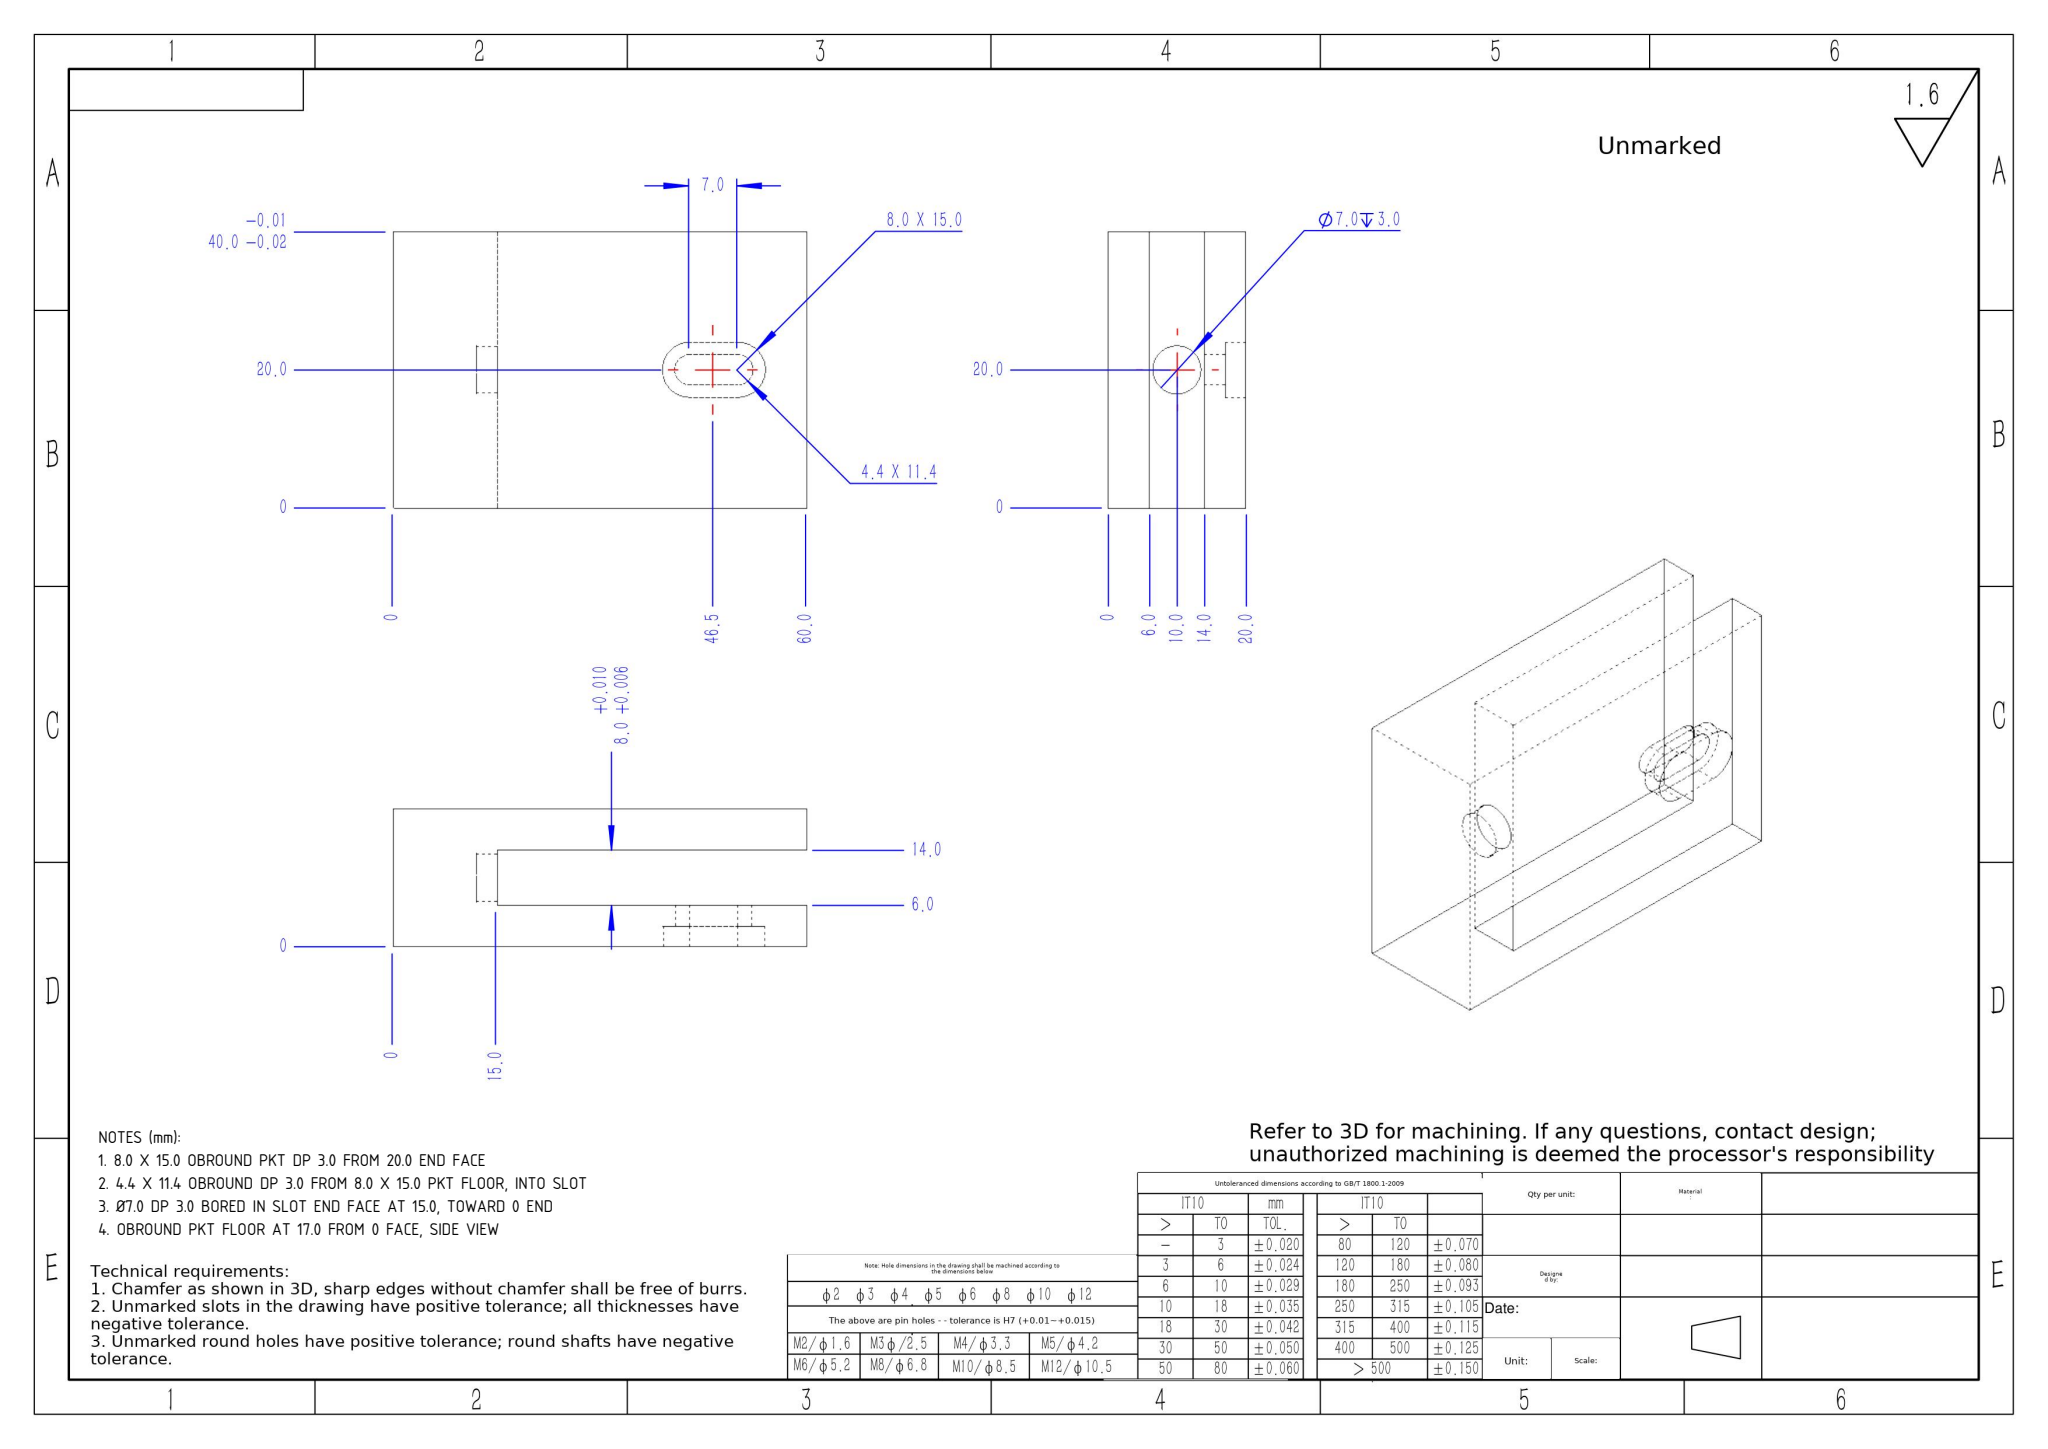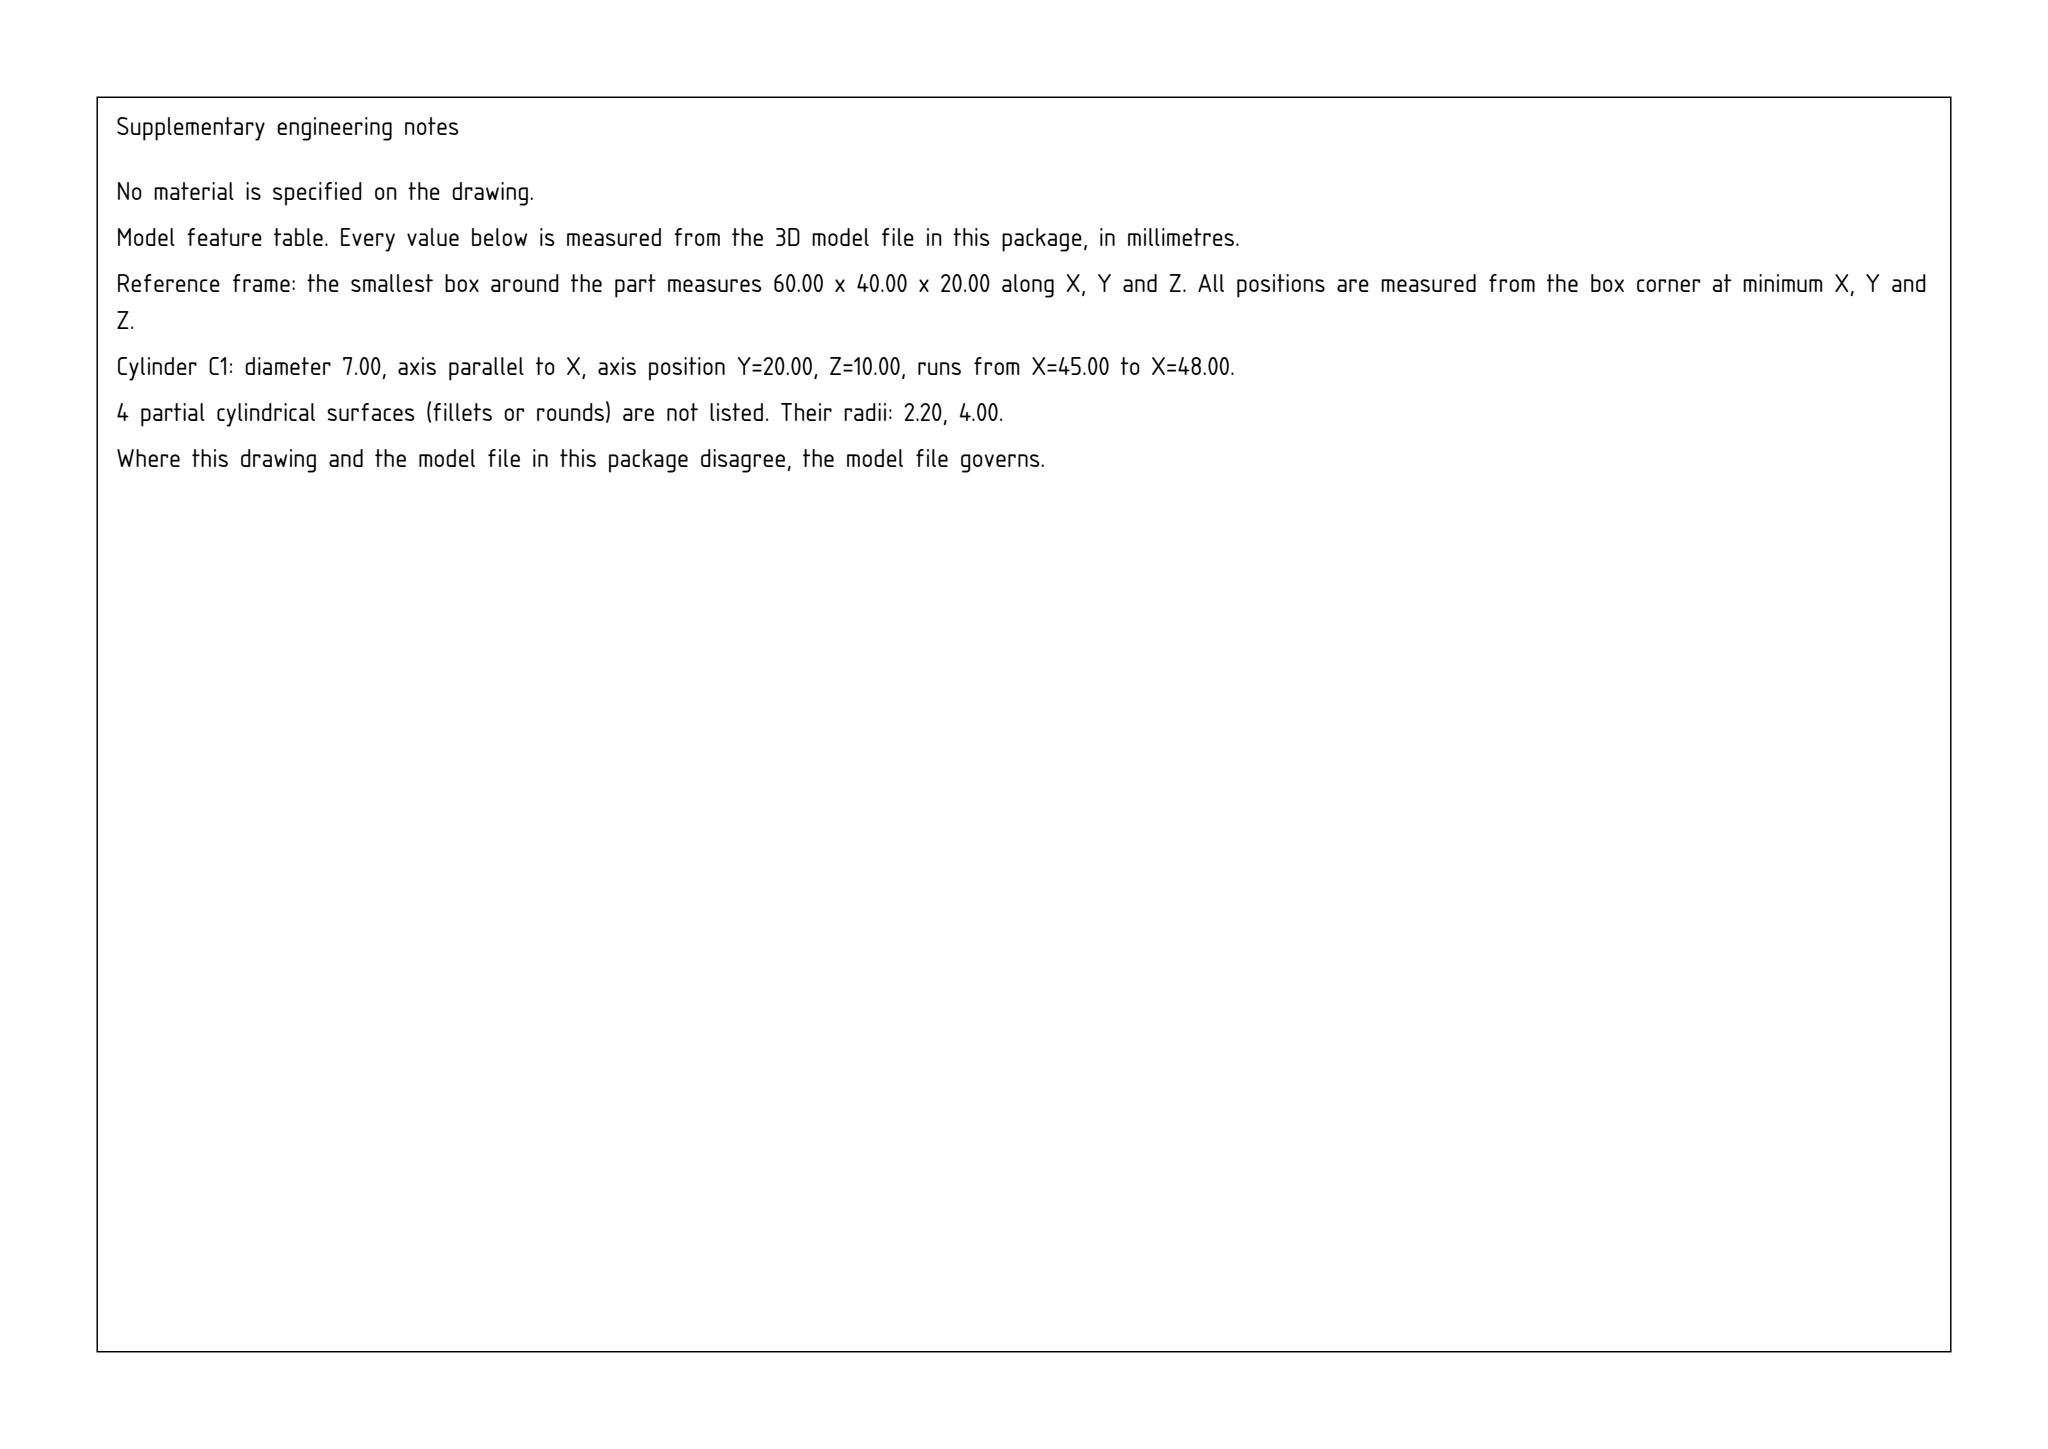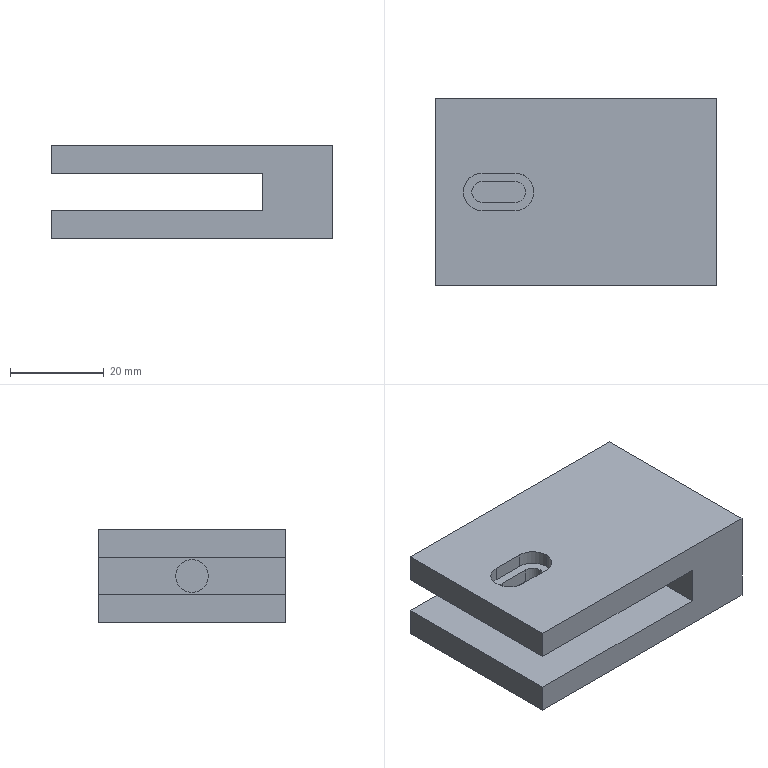Part | SolidWorks | mm | 1 solid | 24 faces | box 60 x 40 x 20 mm | volume 33028 mm3 | plane 16 | cylinder 8 | commonest cylinder face diameters 4.4 x3 8 x3 7 x2
Drawing notes:
8.0 X 15.0 OBROUND PKT DP 3.0 FROM 20.0 END FACE | from the solid: Ø8.0 z-axis cyls at x=10.0 & 17.0, y=20.0, len 3.0; z planes 20.0 & 17.0 (pocket 15.0 long overall = 7.0 ctr dist + 8.0)
4.4 X 11.4 OBROUND DP 3.0 FROM 8.0 X 15.0 PKT FLOOR, INTO SLOT | from the solid: Ø4.4 z-axis cyls at x=10.0 & 17.0, y=20.0, len 3.0; runs z=17.0 to z=14.0, breaking into slot (z planes 6.0/14.0); y planes 17.8/22.2
Ø7.0 DP 3.0 BORED IN SLOT END FACE AT 15.0, TOWARD 0 END | from the solid: Ø7.0 x-axis cyl, y=20.0, z=10.0, len 3.0; x planes 45.0 (slot end face = 15.0 in drawing) and 48.0 (bore btm)
OBROUND PKT FLOOR AT 17.0 FROM 0 FACE, SIDE VIEW | from the solid: z planes at 17.0 and 20.0; Ø8.0/Ø4.4 pocket cyls start at z=20.0 face, 3.0 deep
build123d program:
from build123d import *

# Parameters (mm, degrees)
SKETCH1_W           = 60
SKETCH1_H           = 40
BOSS_EXTRUDE1_DEPTH = 10
SKETCH2_W           = 45
SKETCH2_H           = 8
CUT_EXTRUDE1_DEPTH  = 51.99
CUT_EXTRUDE2_DEPTH  = 3
CUT_EXTRUDE3_DEPTH  = 3
SKETCH5_R           = 3.5
CUT_EXTRUDE4_DEPTH  = 3


with BuildPart() as part:
    # Sketch1 → Boss-Extrude1 (new, symmetric)
    with BuildSketch(Plane.XY):
        Rectangle(SKETCH1_W, SKETCH1_H)
    extrude(amount=BOSS_EXTRUDE1_DEPTH, both=True)

    # Sketch2 → Cut-Extrude1 (cut, through all)
    with BuildSketch(Plane(origin=(0, 20, 0), x_dir=(1, 0, 0), z_dir=(0, 1, 0))):
        with Locations((-7.5, 0)):
            Rectangle(SKETCH2_W, SKETCH2_H)
    extrude(amount=-CUT_EXTRUDE1_DEPTH, mode=Mode.SUBTRACT)

    # Sketch3 → Cut-Extrude2 (cut)
    with BuildSketch(Plane.XY.offset(10)):
        with BuildLine():
            Line((-20, 4), (-13, 4))
            ThreePointArc((-13, 4), (-9, 0), (-13, -4))
            Line((-13, -4), (-20, -4))
            ThreePointArc((-20, -4), (-24, 0), (-20, 4))
        make_face()
    extrude(amount=-CUT_EXTRUDE2_DEPTH, mode=Mode.SUBTRACT)

    # Sketch4 → Cut-Extrude3 (cut)
    with BuildSketch(Plane.XY.offset(7)):
        with BuildLine():
            Line((-20, 2.2), (-13, 2.2))
            ThreePointArc((-13, 2.2), (-10.8, 0), (-13, -2.2))
            Line((-13, -2.2), (-20, -2.2))
            ThreePointArc((-20, -2.2), (-22.2, 0), (-20, 2.2))
        make_face()
    extrude(amount=-CUT_EXTRUDE3_DEPTH, mode=Mode.SUBTRACT)

    # Sketch5 → Cut-Extrude4 (cut)
    with BuildSketch(Plane.ZY.offset(-15)):
        Circle(SKETCH5_R)
    extrude(amount=-CUT_EXTRUDE4_DEPTH, mode=Mode.SUBTRACT)


solid = part.part
STEP:
#1=CARTESIAN_POINT('',(18.,0.,-3.5));
#2=VERTEX_POINT('',#1);
#3=CARTESIAN_POINT('',(18.,0.,3.5));
#4=VERTEX_POINT('',#3);
#5=CARTESIAN_POINT('',(18.,0.,0.));
#6=DIRECTION('',(-1.,0.,0.));
#7=DIRECTION('',(0.,0.,1.));
#8=AXIS2_PLACEMENT_3D('',#5,#6,#7);
#9=CIRCLE('',#8,3.5);
#10=EDGE_CURVE('',#2,#4,#9,.T.);
#11=ORIENTED_EDGE('',*,*,#10,.F.);
#12=CARTESIAN_POINT('',(15.,0.,-3.5));
#13=VERTEX_POINT('',#12);
#14=CARTESIAN_POINT('',(18.,0.,-3.5));
#15=DIRECTION('',(-1.,0.,0.));
#16=VECTOR('',#15,1000.);
#17=LINE('',#14,#16);
#18=EDGE_CURVE('',#2,#13,#17,.T.);
#19=ORIENTED_EDGE('',*,*,#18,.T.);
#20=CARTESIAN_POINT('',(15.,0.,3.5));
#21=VERTEX_POINT('',#20);
#22=CARTESIAN_POINT('',(15.,0.,0.));
#23=DIRECTION('',(-1.,0.,0.));
#24=DIRECTION('',(0.,0.,1.));
#25=AXIS2_PLACEMENT_3D('',#22,#23,#24);
#26=CIRCLE('',#25,3.5);
#27=EDGE_CURVE('',#13,#21,#26,.T.);
#28=ORIENTED_EDGE('',*,*,#27,.T.);
#29=CARTESIAN_POINT('',(18.,0.,3.5));
#30=DIRECTION('',(-1.,0.,0.));
#31=VECTOR('',#30,1000.);
#32=LINE('',#29,#31);
#33=EDGE_CURVE('',#4,#21,#32,.T.);
#34=ORIENTED_EDGE('',*,*,#33,.F.);
#35=EDGE_LOOP('',(#11,#19,#28,#34));
#36=FACE_OUTER_BOUND('',#35,.T.);
#37=CARTESIAN_POINT('',(18.,0.,0.));
#38=DIRECTION('',(-1.,0.,0.));
#39=DIRECTION('',(0.,0.,1.));
#40=AXIS2_PLACEMENT_3D('',#37,#38,#39);
#41=CYLINDRICAL_SURFACE('',#40,3.5);
#42=ADVANCED_FACE('',(#36),#41,.F.);
#43=CARTESIAN_POINT('',(-10.8,0.,4.));
#44=VERTEX_POINT('',#43);
#45=CARTESIAN_POINT('',(-13.,2.2,4.));
#46=VERTEX_POINT('',#45);
#47=CARTESIAN_POINT('',(-13.,0.,4.));
#48=DIRECTION('',(0.,0.,1.));
#49=DIRECTION('',(1.,0.,0.));
#50=AXIS2_PLACEMENT_3D('',#47,#48,#49);
#51=CIRCLE('',#50,2.2);
#52=EDGE_CURVE('',#44,#46,#51,.T.);
#53=ORIENTED_EDGE('',*,*,#52,.F.);
#54=CARTESIAN_POINT('',(-10.8,0.,7.));
#55=VERTEX_POINT('',#54);
#56=CARTESIAN_POINT('',(-10.8,0.,4.));
#57=DIRECTION('',(0.,0.,1.));
#58=VECTOR('',#57,1000.);
#59=LINE('',#56,#58);
#60=EDGE_CURVE('',#44,#55,#59,.T.);
#61=ORIENTED_EDGE('',*,*,#60,.T.);
#62=CARTESIAN_POINT('',(-13.,2.2,7.));
#63=VERTEX_POINT('',#62);
#64=CARTESIAN_POINT('',(-13.,0.,7.));
#65=DIRECTION('',(0.,0.,1.));
#66=DIRECTION('',(1.,0.,0.));
#67=AXIS2_PLACEMENT_3D('',#64,#65,#66);
#68=CIRCLE('',#67,2.2);
#69=EDGE_CURVE('',#55,#63,#68,.T.);
#70=ORIENTED_EDGE('',*,*,#69,.T.);
#71=CARTESIAN_POINT('',(-13.,2.2,4.));
#72=DIRECTION('',(0.,0.,1.));
#73=VECTOR('',#72,1000.);
#74=LINE('',#71,#73);
#75=EDGE_CURVE('',#46,#63,#74,.T.);
#76=ORIENTED_EDGE('',*,*,#75,.F.);
#77=EDGE_LOOP('',(#53,#61,#70,#76));
#78=FACE_OUTER_BOUND('',#77,.T.);
#79=CARTESIAN_POINT('',(-13.,0.,4.));
#80=DIRECTION('',(0.,0.,1.));
#81=DIRECTION('',(1.,0.,0.));
#82=AXIS2_PLACEMENT_3D('',#79,#80,#81);
#83=CYLINDRICAL_SURFACE('',#82,2.2);
#84=ADVANCED_FACE('',(#78),#83,.F.);
#85=CARTESIAN_POINT('',(-9.,0.,7.));
#86=VERTEX_POINT('',#85);
#87=CARTESIAN_POINT('',(-13.,4.,7.));
#88=VERTEX_POINT('',#87);
#89=CARTESIAN_POINT('',(-13.,0.,7.));
#90=DIRECTION('',(0.,0.,1.));
#91=DIRECTION('',(1.,0.,0.));
#92=AXIS2_PLACEMENT_3D('',#89,#90,#91);
#93=CIRCLE('',#92,4.);
#94=EDGE_CURVE('',#86,#88,#93,.T.);
#95=ORIENTED_EDGE('',*,*,#94,.F.);
#96=CARTESIAN_POINT('',(-9.,0.,10.));
#97=VERTEX_POINT('',#96);
#98=CARTESIAN_POINT('',(-9.,0.,7.));
#99=DIRECTION('',(0.,0.,1.));
#100=VECTOR('',#99,1000.);
#101=LINE('',#98,#100);
#102=EDGE_CURVE('',#86,#97,#101,.T.);
#103=ORIENTED_EDGE('',*,*,#102,.T.);
#104=CARTESIAN_POINT('',(-13.,4.,10.));
#105=VERTEX_POINT('',#104);
#106=CARTESIAN_POINT('',(-13.,0.,10.));
#107=DIRECTION('',(0.,0.,1.));
#108=DIRECTION('',(1.,0.,0.));
#109=AXIS2_PLACEMENT_3D('',#106,#107,#108);
#110=CIRCLE('',#109,4.);
#111=EDGE_CURVE('',#97,#105,#110,.T.);
#112=ORIENTED_EDGE('',*,*,#111,.T.);
#113=CARTESIAN_POINT('',(-13.,4.,7.));
#114=DIRECTION('',(0.,0.,1.));
#115=VECTOR('',#114,1000.);
#116=LINE('',#113,#115);
#117=EDGE_CURVE('',#88,#105,#116,.T.);
#118=ORIENTED_EDGE('',*,*,#117,.F.);
#119=EDGE_LOOP('',(#95,#103,#112,#118));
#120=FACE_OUTER_BOUND('',#119,.T.);
#121=CARTESIAN_POINT('',(-13.,0.,7.));
#122=DIRECTION('',(0.,0.,1.));
#123=DIRECTION('',(1.,0.,0.));
#124=AXIS2_PLACEMENT_3D('',#121,#122,#123);
#125=CYLINDRICAL_SURFACE('',#124,4.);
#126=ADVANCED_FACE('',(#120),#125,.F.);
#127=CARTESIAN_POINT('',(-30.,-20.,-4.));
#128=VERTEX_POINT('',#127);
#129=CARTESIAN_POINT('',(-30.,-20.,-10.));
#130=VERTEX_POINT('',#129);
#131=CARTESIAN_POINT('',(-30.,-20.,10.));
#132=DIRECTION('',(0.,0.,-1.));
#133=VECTOR('',#132,1000.);
#134=LINE('',#131,#133);
#135=EDGE_CURVE('',#128,#130,#134,.T.);
#136=ORIENTED_EDGE('',*,*,#135,.F.);
#137=CARTESIAN_POINT('',(-30.,20.,-4.));
#138=VERTEX_POINT('',#137);
#139=CARTESIAN_POINT('',(-30.,-20.,-4.));
#140=DIRECTION('',(0.,1.,0.));
#141=VECTOR('',#140,1000.);
#142=LINE('',#139,#141);
#143=EDGE_CURVE('',#128,#138,#142,.T.);
#144=ORIENTED_EDGE('',*,*,#143,.T.);
#145=CARTESIAN_POINT('',(-30.,20.,-10.));
#146=VERTEX_POINT('',#145);
#147=CARTESIAN_POINT('',(-30.,20.,10.));
#148=DIRECTION('',(0.,0.,-1.));
#149=VECTOR('',#148,1000.);
#150=LINE('',#147,#149);
#151=EDGE_CURVE('',#138,#146,#150,.T.);
#152=ORIENTED_EDGE('',*,*,#151,.T.);
#153=CARTESIAN_POINT('',(-30.,-20.,-10.));
#154=DIRECTION('',(0.,-1.,0.));
#155=VECTOR('',#154,1000.);
#156=LINE('',#153,#155);
#157=EDGE_CURVE('',#146,#130,#156,.T.);
#158=ORIENTED_EDGE('',*,*,#157,.T.);
#159=EDGE_LOOP('',(#136,#144,#152,#158));
#160=FACE_OUTER_BOUND('',#159,.T.);
#161=CARTESIAN_POINT('',(-30.,-20.,10.));
#162=DIRECTION('',(1.,0.,0.));
#163=DIRECTION('',(0.,0.,-1.));
#164=AXIS2_PLACEMENT_3D('',#161,#162,#163);
#165=PLANE('',#164);
#166=ADVANCED_FACE('',(#160),#165,.F.);
#167=CARTESIAN_POINT('',(-30.,20.,10.));
#168=VERTEX_POINT('',#167);
#169=CARTESIAN_POINT('',(-30.,20.,4.));
#170=VERTEX_POINT('',#169);
#171=CARTESIAN_POINT('',(-30.,20.,10.));
#172=DIRECTION('',(0.,0.,-1.));
#173=VECTOR('',#172,1000.);
#174=LINE('',#171,#173);
#175=EDGE_CURVE('',#168,#170,#174,.T.);
#176=ORIENTED_EDGE('',*,*,#175,.T.);
#177=CARTESIAN_POINT('',(-30.,-20.,4.));
#178=VERTEX_POINT('',#177);
#179=CARTESIAN_POINT('',(-30.,-20.,4.));
#180=DIRECTION('',(0.,1.,0.));
#181=VECTOR('',#180,1000.);
#182=LINE('',#179,#181);
#183=EDGE_CURVE('',#178,#170,#182,.T.);
#184=ORIENTED_EDGE('',*,*,#183,.F.);
#185=CARTESIAN_POINT('',(-30.,-20.,10.));
#186=VERTEX_POINT('',#185);
#187=CARTESIAN_POINT('',(-30.,-20.,10.));
#188=DIRECTION('',(0.,0.,-1.));
#189=VECTOR('',#188,1000.);
#190=LINE('',#187,#189);
#191=EDGE_CURVE('',#186,#178,#190,.T.);
#192=ORIENTED_EDGE('',*,*,#191,.F.);
#193=CARTESIAN_POINT('',(-30.,-20.,10.));
#194=DIRECTION('',(0.,-1.,0.));
#195=VECTOR('',#194,1000.);
#196=LINE('',#193,#195);
#197=EDGE_CURVE('',#168,#186,#196,.T.);
#198=ORIENTED_EDGE('',*,*,#197,.F.);
#199=EDGE_LOOP('',(#176,#184,#192,#198));
#200=FACE_OUTER_BOUND('',#199,.T.);
#201=CARTESIAN_POINT('',(-30.,-20.,10.));
#202=DIRECTION('',(1.,0.,0.));
#203=DIRECTION('',(0.,0.,-1.));
#204=AXIS2_PLACEMENT_3D('',#201,#202,#203);
#205=PLANE('',#204);
#206=ADVANCED_FACE('',(#200),#205,.F.);
#207=CARTESIAN_POINT('',(15.,-20.,4.));
#208=VERTEX_POINT('',#207);
#209=CARTESIAN_POINT('',(15.,-20.,-4.));
#210=VERTEX_POINT('',#209);
#211=CARTESIAN_POINT('',(15.,-20.,-4.));
#212=DIRECTION('',(0.,0.,-1.));
#213=VECTOR('',#212,1000.);
#214=LINE('',#211,#213);
#215=EDGE_CURVE('',#208,#210,#214,.T.);
#216=ORIENTED_EDGE('',*,*,#215,.T.);
#217=CARTESIAN_POINT('',(-30.,-20.,-4.));
#218=DIRECTION('',(-1.,0.,0.));
#219=VECTOR('',#218,1000.);
#220=LINE('',#217,#219);
#221=EDGE_CURVE('',#210,#128,#220,.T.);
#222=ORIENTED_EDGE('',*,*,#221,.T.);
#223=ORIENTED_EDGE('',*,*,#135,.T.);
#224=CARTESIAN_POINT('',(30.,-20.,-10.));
#225=VERTEX_POINT('',#224);
#226=CARTESIAN_POINT('',(30.,-20.,-10.));
#227=DIRECTION('',(1.,-0.,0.));
#228=VECTOR('',#227,1000.);
#229=LINE('',#226,#228);
#230=EDGE_CURVE('',#130,#225,#229,.T.);
#231=ORIENTED_EDGE('',*,*,#230,.T.);
#232=CARTESIAN_POINT('',(30.,-20.,10.));
#233=VERTEX_POINT('',#232);
#234=CARTESIAN_POINT('',(30.,-20.,10.));
#235=DIRECTION('',(0.,0.,-1.));
#236=VECTOR('',#235,1000.);
#237=LINE('',#234,#236);
#238=EDGE_CURVE('',#233,#225,#237,.T.);
#239=ORIENTED_EDGE('',*,*,#238,.F.);
#240=CARTESIAN_POINT('',(30.,-20.,10.));
#241=DIRECTION('',(1.,-0.,0.));
#242=VECTOR('',#241,1000.);
#243=LINE('',#240,#242);
#244=EDGE_CURVE('',#186,#233,#243,.T.);
#245=ORIENTED_EDGE('',*,*,#244,.F.);
#246=ORIENTED_EDGE('',*,*,#191,.T.);
#247=CARTESIAN_POINT('',(-30.,-20.,4.));
#248=DIRECTION('',(1.,0.,0.));
#249=VECTOR('',#248,1000.);
#250=LINE('',#247,#249);
#251=EDGE_CURVE('',#178,#208,#250,.T.);
#252=ORIENTED_EDGE('',*,*,#251,.T.);
#253=EDGE_LOOP('',(#216,#222,#223,#231,#239,#245,#246,#252));
#254=FACE_OUTER_BOUND('',#253,.T.);
#255=CARTESIAN_POINT('',(30.,-20.,10.));
#256=DIRECTION('',(0.,1.,0.));
#257=DIRECTION('',(-1.,0.,0.));
#258=AXIS2_PLACEMENT_3D('',#255,#256,#257);
#259=PLANE('',#258);
#260=ADVANCED_FACE('',(#254),#259,.F.);
#261=CARTESIAN_POINT('',(30.,20.,-10.));
#262=VERTEX_POINT('',#261);
#263=CARTESIAN_POINT('',(30.,-20.,-10.));
#264=DIRECTION('',(-0.,1.,0.));
#265=VECTOR('',#264,1000.);
#266=LINE('',#263,#265);
#267=EDGE_CURVE('',#225,#262,#266,.T.);
#268=ORIENTED_EDGE('',*,*,#267,.T.);
#269=CARTESIAN_POINT('',(30.,20.,10.));
#270=VERTEX_POINT('',#269);
#271=CARTESIAN_POINT('',(30.,20.,10.));
#272=DIRECTION('',(0.,0.,-1.));
#273=VECTOR('',#272,1000.);
#274=LINE('',#271,#273);
#275=EDGE_CURVE('',#270,#262,#274,.T.);
#276=ORIENTED_EDGE('',*,*,#275,.F.);
#277=CARTESIAN_POINT('',(30.,-20.,10.));
#278=DIRECTION('',(-0.,1.,0.));
#279=VECTOR('',#278,1000.);
#280=LINE('',#277,#279);
#281=EDGE_CURVE('',#233,#270,#280,.T.);
#282=ORIENTED_EDGE('',*,*,#281,.F.);
#283=ORIENTED_EDGE('',*,*,#238,.T.);
#284=EDGE_LOOP('',(#268,#276,#282,#283));
#285=FACE_OUTER_BOUND('',#284,.T.);
#286=CARTESIAN_POINT('',(30.,-20.,10.));
#287=DIRECTION('',(-1.,-0.,0.));
#288=DIRECTION('',(0.,-1.,0.));
#289=AXIS2_PLACEMENT_3D('',#286,#287,#288);
#290=PLANE('',#289);
#291=ADVANCED_FACE('',(#285),#290,.F.);
#292=ORIENTED_EDGE('',*,*,#151,.F.);
#293=CARTESIAN_POINT('',(15.,20.,-4.));
#294=VERTEX_POINT('',#293);
#295=CARTESIAN_POINT('',(-30.,20.,-4.));
#296=DIRECTION('',(-1.,0.,0.));
#297=VECTOR('',#296,1000.);
#298=LINE('',#295,#297);
#299=EDGE_CURVE('',#294,#138,#298,.T.);
#300=ORIENTED_EDGE('',*,*,#299,.F.);
#301=CARTESIAN_POINT('',(15.,20.,4.));
#302=VERTEX_POINT('',#301);
#303=CARTESIAN_POINT('',(15.,20.,-4.));
#304=DIRECTION('',(0.,0.,-1.));
#305=VECTOR('',#304,1000.);
#306=LINE('',#303,#305);
#307=EDGE_CURVE('',#302,#294,#306,.T.);
#308=ORIENTED_EDGE('',*,*,#307,.F.);
#309=CARTESIAN_POINT('',(-30.,20.,4.));
#310=DIRECTION('',(1.,0.,0.));
#311=VECTOR('',#310,1000.);
#312=LINE('',#309,#311);
#313=EDGE_CURVE('',#170,#302,#312,.T.);
#314=ORIENTED_EDGE('',*,*,#313,.F.);
#315=ORIENTED_EDGE('',*,*,#175,.F.);
#316=CARTESIAN_POINT('',(30.,20.,10.));
#317=DIRECTION('',(-1.,0.,0.));
#318=VECTOR('',#317,1000.);
#319=LINE('',#316,#318);
#320=EDGE_CURVE('',#270,#168,#319,.T.);
#321=ORIENTED_EDGE('',*,*,#320,.F.);
#322=ORIENTED_EDGE('',*,*,#275,.T.);
#323=CARTESIAN_POINT('',(30.,20.,-10.));
#324=DIRECTION('',(-1.,0.,0.));
#325=VECTOR('',#324,1000.);
#326=LINE('',#323,#325);
#327=EDGE_CURVE('',#262,#146,#326,.T.);
#328=ORIENTED_EDGE('',*,*,#327,.T.);
#329=EDGE_LOOP('',(#292,#300,#308,#314,#315,#321,#322,#328));
#330=FACE_OUTER_BOUND('',#329,.T.);
#331=CARTESIAN_POINT('',(30.,20.,10.));
#332=DIRECTION('',(0.,-1.,0.));
#333=DIRECTION('',(0.,0.,-1.));
#334=AXIS2_PLACEMENT_3D('',#331,#332,#333);
#335=PLANE('',#334);
#336=ADVANCED_FACE('',(#330),#335,.F.);
#337=CARTESIAN_POINT('',(-20.,4.,10.));
#338=VERTEX_POINT('',#337);
#339=CARTESIAN_POINT('',(-20.,-4.,10.));
#340=VERTEX_POINT('',#339);
#341=CARTESIAN_POINT('',(-20.,0.,10.));
#342=DIRECTION('',(0.,0.,1.));
#343=DIRECTION('',(1.,0.,0.));
#344=AXIS2_PLACEMENT_3D('',#341,#342,#343);
#345=CIRCLE('',#344,4.);
#346=EDGE_CURVE('',#338,#340,#345,.T.);
#347=ORIENTED_EDGE('',*,*,#346,.F.);
#348=CARTESIAN_POINT('',(-20.,4.,10.));
#349=DIRECTION('',(-1.,0.,0.));
#350=VECTOR('',#349,1000.);
#351=LINE('',#348,#350);
#352=EDGE_CURVE('',#105,#338,#351,.T.);
#353=ORIENTED_EDGE('',*,*,#352,.F.);
#354=ORIENTED_EDGE('',*,*,#111,.F.);
#355=CARTESIAN_POINT('',(-13.,-4.,10.));
#356=VERTEX_POINT('',#355);
#357=CARTESIAN_POINT('',(-13.,0.,10.));
#358=DIRECTION('',(0.,0.,1.));
#359=DIRECTION('',(1.,0.,0.));
#360=AXIS2_PLACEMENT_3D('',#357,#358,#359);
#361=CIRCLE('',#360,4.);
#362=EDGE_CURVE('',#356,#97,#361,.T.);
#363=ORIENTED_EDGE('',*,*,#362,.F.);
#364=CARTESIAN_POINT('',(-20.,-4.,10.));
#365=DIRECTION('',(1.,0.,0.));
#366=VECTOR('',#365,1000.);
#367=LINE('',#364,#366);
#368=EDGE_CURVE('',#340,#356,#367,.T.);
#369=ORIENTED_EDGE('',*,*,#368,.F.);
#370=EDGE_LOOP('',(#347,#353,#354,#363,#369));
#371=FACE_BOUND('',#370,.T.);
#372=ORIENTED_EDGE('',*,*,#197,.T.);
#373=ORIENTED_EDGE('',*,*,#244,.T.);
#374=ORIENTED_EDGE('',*,*,#281,.T.);
#375=ORIENTED_EDGE('',*,*,#320,.T.);
#376=EDGE_LOOP('',(#372,#373,#374,#375));
#377=FACE_OUTER_BOUND('',#376,.T.);
#378=CARTESIAN_POINT('',(0.,0.,10.));
#379=DIRECTION('',(0.,0.,1.));
#380=DIRECTION('',(1.,0.,0.));
#381=AXIS2_PLACEMENT_3D('',#378,#379,#380);
#382=PLANE('',#381);
#383=ADVANCED_FACE('',(#371,#377),#382,.T.);
#384=ORIENTED_EDGE('',*,*,#157,.F.);
#385=ORIENTED_EDGE('',*,*,#327,.F.);
#386=ORIENTED_EDGE('',*,*,#267,.F.);
#387=ORIENTED_EDGE('',*,*,#230,.F.);
#388=EDGE_LOOP('',(#384,#385,#386,#387));
#389=FACE_OUTER_BOUND('',#388,.T.);
#390=CARTESIAN_POINT('',(0.,0.,-10.));
#391=DIRECTION('',(0.,0.,1.));
#392=DIRECTION('',(1.,0.,0.));
#393=AXIS2_PLACEMENT_3D('',#390,#391,#392);
#394=PLANE('',#393);
#395=ADVANCED_FACE('',(#389),#394,.F.);
#396=ORIENTED_EDGE('',*,*,#299,.T.);
#397=ORIENTED_EDGE('',*,*,#143,.F.);
#398=ORIENTED_EDGE('',*,*,#221,.F.);
#399=CARTESIAN_POINT('',(15.,-20.,-4.));
#400=DIRECTION('',(0.,1.,0.));
#401=VECTOR('',#400,1000.);
#402=LINE('',#399,#401);
#403=EDGE_CURVE('',#210,#294,#402,.T.);
#404=ORIENTED_EDGE('',*,*,#403,.T.);
#405=EDGE_LOOP('',(#396,#397,#398,#404));
#406=FACE_OUTER_BOUND('',#405,.T.);
#407=CARTESIAN_POINT('',(-30.,-20.,-4.));
#408=DIRECTION('',(0.,0.,-1.));
#409=DIRECTION('',(-1.,0.,0.));
#410=AXIS2_PLACEMENT_3D('',#407,#408,#409);
#411=PLANE('',#410);
#412=ADVANCED_FACE('',(#406),#411,.F.);
#413=CARTESIAN_POINT('',(15.,0.,0.));
#414=DIRECTION('',(-1.,0.,0.));
#415=DIRECTION('',(0.,0.,1.));
#416=AXIS2_PLACEMENT_3D('',#413,#414,#415);
#417=CIRCLE('',#416,3.5);
#418=EDGE_CURVE('',#21,#13,#417,.T.);
#419=ORIENTED_EDGE('',*,*,#418,.F.);
#420=ORIENTED_EDGE('',*,*,#27,.F.);
#421=EDGE_LOOP('',(#419,#420));
#422=FACE_BOUND('',#421,.T.);
#423=ORIENTED_EDGE('',*,*,#307,.T.);
#424=ORIENTED_EDGE('',*,*,#403,.F.);
#425=ORIENTED_EDGE('',*,*,#215,.F.);
#426=CARTESIAN_POINT('',(15.,-20.,4.));
#427=DIRECTION('',(0.,1.,0.));
#428=VECTOR('',#427,1000.);
#429=LINE('',#426,#428);
#430=EDGE_CURVE('',#208,#302,#429,.T.);
#431=ORIENTED_EDGE('',*,*,#430,.T.);
#432=EDGE_LOOP('',(#423,#424,#425,#431));
#433=FACE_OUTER_BOUND('',#432,.T.);
#434=CARTESIAN_POINT('',(15.,-20.,-4.));
#435=DIRECTION('',(1.,0.,0.));
#436=DIRECTION('',(0.,0.,-1.));
#437=AXIS2_PLACEMENT_3D('',#434,#435,#436);
#438=PLANE('',#437);
#439=ADVANCED_FACE('',(#422,#433),#438,.F.);
#440=CARTESIAN_POINT('',(-20.,2.2,4.));
#441=VERTEX_POINT('',#440);
#442=CARTESIAN_POINT('',(-20.,2.2,4.));
#443=DIRECTION('',(-1.,0.,0.));
#444=VECTOR('',#443,1000.);
#445=LINE('',#442,#444);
#446=EDGE_CURVE('',#46,#441,#445,.T.);
#447=ORIENTED_EDGE('',*,*,#446,.T.);
#448=CARTESIAN_POINT('',(-20.,-2.2,4.));
#449=VERTEX_POINT('',#448);
#450=CARTESIAN_POINT('',(-20.,0.,4.));
#451=DIRECTION('',(0.,0.,1.));
#452=DIRECTION('',(1.,0.,0.));
#453=AXIS2_PLACEMENT_3D('',#450,#451,#452);
#454=CIRCLE('',#453,2.2);
#455=EDGE_CURVE('',#441,#449,#454,.T.);
#456=ORIENTED_EDGE('',*,*,#455,.T.);
#457=CARTESIAN_POINT('',(-13.,-2.2,4.));
#458=VERTEX_POINT('',#457);
#459=CARTESIAN_POINT('',(-20.,-2.2,4.));
#460=DIRECTION('',(1.,0.,0.));
#461=VECTOR('',#460,1000.);
#462=LINE('',#459,#461);
#463=EDGE_CURVE('',#449,#458,#462,.T.);
#464=ORIENTED_EDGE('',*,*,#463,.T.);
#465=CARTESIAN_POINT('',(-13.,0.,4.));
#466=DIRECTION('',(0.,0.,1.));
#467=DIRECTION('',(1.,0.,0.));
#468=AXIS2_PLACEMENT_3D('',#465,#466,#467);
#469=CIRCLE('',#468,2.2);
#470=EDGE_CURVE('',#458,#44,#469,.T.);
#471=ORIENTED_EDGE('',*,*,#470,.T.);
#472=ORIENTED_EDGE('',*,*,#52,.T.);
#473=EDGE_LOOP('',(#447,#456,#464,#471,#472));
#474=FACE_BOUND('',#473,.T.);
#475=ORIENTED_EDGE('',*,*,#313,.T.);
#476=ORIENTED_EDGE('',*,*,#430,.F.);
#477=ORIENTED_EDGE('',*,*,#251,.F.);
#478=ORIENTED_EDGE('',*,*,#183,.T.);
#479=EDGE_LOOP('',(#475,#476,#477,#478));
#480=FACE_OUTER_BOUND('',#479,.T.);
#481=CARTESIAN_POINT('',(-30.,-20.,4.));
#482=DIRECTION('',(0.,0.,1.));
#483=DIRECTION('',(1.,0.,0.));
#484=AXIS2_PLACEMENT_3D('',#481,#482,#483);
#485=PLANE('',#484);
#486=ADVANCED_FACE('',(#474,#480),#485,.F.);
#487=ORIENTED_EDGE('',*,*,#346,.T.);
#488=CARTESIAN_POINT('',(-20.,-4.,7.));
#489=VERTEX_POINT('',#488);
#490=CARTESIAN_POINT('',(-20.,-4.,7.));
#491=DIRECTION('',(0.,0.,1.));
#492=VECTOR('',#491,1000.);
#493=LINE('',#490,#492);
#494=EDGE_CURVE('',#489,#340,#493,.T.);
#495=ORIENTED_EDGE('',*,*,#494,.F.);
#496=CARTESIAN_POINT('',(-20.,4.,7.));
#497=VERTEX_POINT('',#496);
#498=CARTESIAN_POINT('',(-20.,0.,7.));
#499=DIRECTION('',(0.,0.,1.));
#500=DIRECTION('',(1.,0.,0.));
#501=AXIS2_PLACEMENT_3D('',#498,#499,#500);
#502=CIRCLE('',#501,4.);
#503=EDGE_CURVE('',#497,#489,#502,.T.);
#504=ORIENTED_EDGE('',*,*,#503,.F.);
#505=CARTESIAN_POINT('',(-20.,4.,7.));
#506=DIRECTION('',(0.,0.,1.));
#507=VECTOR('',#506,1000.);
#508=LINE('',#505,#507);
#509=EDGE_CURVE('',#497,#338,#508,.T.);
#510=ORIENTED_EDGE('',*,*,#509,.T.);
#511=EDGE_LOOP('',(#487,#495,#504,#510));
#512=FACE_OUTER_BOUND('',#511,.T.);
#513=CARTESIAN_POINT('',(-20.,0.,7.));
#514=DIRECTION('',(0.,0.,1.));
#515=DIRECTION('',(1.,0.,0.));
#516=AXIS2_PLACEMENT_3D('',#513,#514,#515);
#517=CYLINDRICAL_SURFACE('',#516,4.);
#518=ADVANCED_FACE('',(#512),#517,.F.);
#519=ORIENTED_EDGE('',*,*,#352,.T.);
#520=ORIENTED_EDGE('',*,*,#509,.F.);
#521=CARTESIAN_POINT('',(-20.,4.,7.));
#522=DIRECTION('',(-1.,0.,0.));
#523=VECTOR('',#522,1000.);
#524=LINE('',#521,#523);
#525=EDGE_CURVE('',#88,#497,#524,.T.);
#526=ORIENTED_EDGE('',*,*,#525,.F.);
#527=ORIENTED_EDGE('',*,*,#117,.T.);
#528=EDGE_LOOP('',(#519,#520,#526,#527));
#529=FACE_OUTER_BOUND('',#528,.T.);
#530=CARTESIAN_POINT('',(-20.,4.,7.));
#531=DIRECTION('',(0.,1.,0.));
#532=DIRECTION('',(0.,0.,1.));
#533=AXIS2_PLACEMENT_3D('',#530,#531,#532);
#534=PLANE('',#533);
#535=ADVANCED_FACE('',(#529),#534,.F.);
#536=ORIENTED_EDGE('',*,*,#102,.F.);
#537=CARTESIAN_POINT('',(-13.,-4.,7.));
#538=VERTEX_POINT('',#537);
#539=CARTESIAN_POINT('',(-13.,0.,7.));
#540=DIRECTION('',(0.,0.,1.));
#541=DIRECTION('',(1.,0.,0.));
#542=AXIS2_PLACEMENT_3D('',#539,#540,#541);
#543=CIRCLE('',#542,4.);
#544=EDGE_CURVE('',#538,#86,#543,.T.);
#545=ORIENTED_EDGE('',*,*,#544,.F.);
#546=CARTESIAN_POINT('',(-13.,-4.,7.));
#547=DIRECTION('',(0.,0.,1.));
#548=VECTOR('',#547,1000.);
#549=LINE('',#546,#548);
#550=EDGE_CURVE('',#538,#356,#549,.T.);
#551=ORIENTED_EDGE('',*,*,#550,.T.);
#552=ORIENTED_EDGE('',*,*,#362,.T.);
#553=EDGE_LOOP('',(#536,#545,#551,#552));
#554=FACE_OUTER_BOUND('',#553,.T.);
#555=CARTESIAN_POINT('',(-13.,0.,7.));
#556=DIRECTION('',(0.,0.,1.));
#557=DIRECTION('',(1.,0.,0.));
#558=AXIS2_PLACEMENT_3D('',#555,#556,#557);
#559=CYLINDRICAL_SURFACE('',#558,4.);
#560=ADVANCED_FACE('',(#554),#559,.F.);
#561=ORIENTED_EDGE('',*,*,#368,.T.);
#562=ORIENTED_EDGE('',*,*,#550,.F.);
#563=CARTESIAN_POINT('',(-20.,-4.,7.));
#564=DIRECTION('',(1.,0.,0.));
#565=VECTOR('',#564,1000.);
#566=LINE('',#563,#565);
#567=EDGE_CURVE('',#489,#538,#566,.T.);
#568=ORIENTED_EDGE('',*,*,#567,.F.);
#569=ORIENTED_EDGE('',*,*,#494,.T.);
#570=EDGE_LOOP('',(#561,#562,#568,#569));
#571=FACE_OUTER_BOUND('',#570,.T.);
#572=CARTESIAN_POINT('',(-20.,-4.,7.));
#573=DIRECTION('',(0.,-1.,0.));
#574=DIRECTION('',(0.,0.,-1.));
#575=AXIS2_PLACEMENT_3D('',#572,#573,#574);
#576=PLANE('',#575);
#577=ADVANCED_FACE('',(#571),#576,.F.);
#578=CARTESIAN_POINT('',(-20.,2.2,7.));
#579=VERTEX_POINT('',#578);
#580=CARTESIAN_POINT('',(-20.,-2.2,7.));
#581=VERTEX_POINT('',#580);
#582=CARTESIAN_POINT('',(-20.,0.,7.));
#583=DIRECTION('',(0.,0.,1.));
#584=DIRECTION('',(1.,0.,0.));
#585=AXIS2_PLACEMENT_3D('',#582,#583,#584);
#586=CIRCLE('',#585,2.2);
#587=EDGE_CURVE('',#579,#581,#586,.T.);
#588=ORIENTED_EDGE('',*,*,#587,.F.);
#589=CARTESIAN_POINT('',(-20.,2.2,7.));
#590=DIRECTION('',(-1.,0.,0.));
#591=VECTOR('',#590,1000.);
#592=LINE('',#589,#591);
#593=EDGE_CURVE('',#63,#579,#592,.T.);
#594=ORIENTED_EDGE('',*,*,#593,.F.);
#595=ORIENTED_EDGE('',*,*,#69,.F.);
#596=CARTESIAN_POINT('',(-13.,-2.2,7.));
#597=VERTEX_POINT('',#596);
#598=CARTESIAN_POINT('',(-13.,0.,7.));
#599=DIRECTION('',(0.,0.,1.));
#600=DIRECTION('',(1.,0.,0.));
#601=AXIS2_PLACEMENT_3D('',#598,#599,#600);
#602=CIRCLE('',#601,2.2);
#603=EDGE_CURVE('',#597,#55,#602,.T.);
#604=ORIENTED_EDGE('',*,*,#603,.F.);
#605=CARTESIAN_POINT('',(-20.,-2.2,7.));
#606=DIRECTION('',(1.,0.,0.));
#607=VECTOR('',#606,1000.);
#608=LINE('',#605,#607);
#609=EDGE_CURVE('',#581,#597,#608,.T.);
#610=ORIENTED_EDGE('',*,*,#609,.F.);
#611=EDGE_LOOP('',(#588,#594,#595,#604,#610));
#612=FACE_BOUND('',#611,.T.);
#613=ORIENTED_EDGE('',*,*,#503,.T.);
#614=ORIENTED_EDGE('',*,*,#567,.T.);
#615=ORIENTED_EDGE('',*,*,#544,.T.);
#616=ORIENTED_EDGE('',*,*,#94,.T.);
#617=ORIENTED_EDGE('',*,*,#525,.T.);
#618=EDGE_LOOP('',(#613,#614,#615,#616,#617));
#619=FACE_OUTER_BOUND('',#618,.T.);
#620=CARTESIAN_POINT('',(-20.,0.,7.));
#621=DIRECTION('',(0.,0.,1.));
#622=DIRECTION('',(1.,0.,0.));
#623=AXIS2_PLACEMENT_3D('',#620,#621,#622);
#624=PLANE('',#623);
#625=ADVANCED_FACE('',(#612,#619),#624,.T.);
#626=ORIENTED_EDGE('',*,*,#587,.T.);
#627=CARTESIAN_POINT('',(-20.,-2.2,4.));
#628=DIRECTION('',(0.,0.,1.));
#629=VECTOR('',#628,1000.);
#630=LINE('',#627,#629);
#631=EDGE_CURVE('',#449,#581,#630,.T.);
#632=ORIENTED_EDGE('',*,*,#631,.F.);
#633=ORIENTED_EDGE('',*,*,#455,.F.);
#634=CARTESIAN_POINT('',(-20.,2.2,4.));
#635=DIRECTION('',(0.,0.,1.));
#636=VECTOR('',#635,1000.);
#637=LINE('',#634,#636);
#638=EDGE_CURVE('',#441,#579,#637,.T.);
#639=ORIENTED_EDGE('',*,*,#638,.T.);
#640=EDGE_LOOP('',(#626,#632,#633,#639));
#641=FACE_OUTER_BOUND('',#640,.T.);
#642=CARTESIAN_POINT('',(-20.,0.,4.));
#643=DIRECTION('',(0.,0.,1.));
#644=DIRECTION('',(1.,0.,0.));
#645=AXIS2_PLACEMENT_3D('',#642,#643,#644);
#646=CYLINDRICAL_SURFACE('',#645,2.2);
#647=ADVANCED_FACE('',(#641),#646,.F.);
#648=ORIENTED_EDGE('',*,*,#593,.T.);
#649=ORIENTED_EDGE('',*,*,#638,.F.);
#650=ORIENTED_EDGE('',*,*,#446,.F.);
#651=ORIENTED_EDGE('',*,*,#75,.T.);
#652=EDGE_LOOP('',(#648,#649,#650,#651));
#653=FACE_OUTER_BOUND('',#652,.T.);
#654=CARTESIAN_POINT('',(-20.,2.2,4.));
#655=DIRECTION('',(0.,1.,0.));
#656=DIRECTION('',(0.,0.,1.));
#657=AXIS2_PLACEMENT_3D('',#654,#655,#656);
#658=PLANE('',#657);
#659=ADVANCED_FACE('',(#653),#658,.F.);
#660=ORIENTED_EDGE('',*,*,#60,.F.);
#661=ORIENTED_EDGE('',*,*,#470,.F.);
#662=CARTESIAN_POINT('',(-13.,-2.2,4.));
#663=DIRECTION('',(0.,0.,1.));
#664=VECTOR('',#663,1000.);
#665=LINE('',#662,#664);
#666=EDGE_CURVE('',#458,#597,#665,.T.);
#667=ORIENTED_EDGE('',*,*,#666,.T.);
#668=ORIENTED_EDGE('',*,*,#603,.T.);
#669=EDGE_LOOP('',(#660,#661,#667,#668));
#670=FACE_OUTER_BOUND('',#669,.T.);
#671=CARTESIAN_POINT('',(-13.,0.,4.));
#672=DIRECTION('',(0.,0.,1.));
#673=DIRECTION('',(1.,0.,0.));
#674=AXIS2_PLACEMENT_3D('',#671,#672,#673);
#675=CYLINDRICAL_SURFACE('',#674,2.2);
#676=ADVANCED_FACE('',(#670),#675,.F.);
#677=ORIENTED_EDGE('',*,*,#609,.T.);
#678=ORIENTED_EDGE('',*,*,#666,.F.);
#679=ORIENTED_EDGE('',*,*,#463,.F.);
#680=ORIENTED_EDGE('',*,*,#631,.T.);
#681=EDGE_LOOP('',(#677,#678,#679,#680));
#682=FACE_OUTER_BOUND('',#681,.T.);
#683=CARTESIAN_POINT('',(-20.,-2.2,4.));
#684=DIRECTION('',(0.,-1.,0.));
#685=DIRECTION('',(0.,0.,-1.));
#686=AXIS2_PLACEMENT_3D('',#683,#684,#685);
#687=PLANE('',#686);
#688=ADVANCED_FACE('',(#682),#687,.F.);
#689=ORIENTED_EDGE('',*,*,#18,.F.);
#690=CARTESIAN_POINT('',(18.,0.,0.));
#691=DIRECTION('',(-1.,0.,0.));
#692=DIRECTION('',(0.,0.,1.));
#693=AXIS2_PLACEMENT_3D('',#690,#691,#692);
#694=CIRCLE('',#693,3.5);
#695=EDGE_CURVE('',#4,#2,#694,.T.);
#696=ORIENTED_EDGE('',*,*,#695,.F.);
#697=ORIENTED_EDGE('',*,*,#33,.T.);
#698=ORIENTED_EDGE('',*,*,#418,.T.);
#699=EDGE_LOOP('',(#689,#696,#697,#698));
#700=FACE_OUTER_BOUND('',#699,.T.);
#701=CARTESIAN_POINT('',(18.,0.,0.));
#702=DIRECTION('',(-1.,0.,0.));
#703=DIRECTION('',(0.,0.,1.));
#704=AXIS2_PLACEMENT_3D('',#701,#702,#703);
#705=CYLINDRICAL_SURFACE('',#704,3.5);
#706=ADVANCED_FACE('',(#700),#705,.F.);
#707=ORIENTED_EDGE('',*,*,#695,.T.);
#708=ORIENTED_EDGE('',*,*,#10,.T.);
#709=EDGE_LOOP('',(#707,#708));
#710=FACE_OUTER_BOUND('',#709,.T.);
#711=CARTESIAN_POINT('',(18.,0.,0.));
#712=DIRECTION('',(-1.,0.,0.));
#713=DIRECTION('',(0.,0.,1.));
#714=AXIS2_PLACEMENT_3D('',#711,#712,#713);
#715=PLANE('',#714);
#716=ADVANCED_FACE('',(#710),#715,.T.);
#717=CLOSED_SHELL('',(#42,#84,#126,#166,#206,#260,#291,#336,#383,#395,#412,#439,#486,#518,#535,#560,#577,#625,#647,#659,#676,#688,#706,#716));
#718=MANIFOLD_SOLID_BREP('',#717);
#719=CARTESIAN_POINT('',(0.,0.,0.));
#720=DIRECTION('',(0.,0.,1.));
#721=DIRECTION('',(1.,0.,0.));
#722=AXIS2_PLACEMENT_3D('',#719,#720,#721);
#723=(LENGTH_UNIT()NAMED_UNIT(*)SI_UNIT(.MILLI.,.METRE.));
#724=UNCERTAINTY_MEASURE_WITH_UNIT(LENGTH_MEASURE(0.00001),#723,'','');
#725=(NAMED_UNIT(*)PLANE_ANGLE_UNIT()SI_UNIT($,.RADIAN.));
#726=(NAMED_UNIT(*)SI_UNIT($,.STERADIAN.)SOLID_ANGLE_UNIT());
#727=(GEOMETRIC_REPRESENTATION_CONTEXT(3)GLOBAL_UNCERTAINTY_ASSIGNED_CONTEXT((#724))GLOBAL_UNIT_ASSIGNED_CONTEXT((#723,#725,#726))REPRESENTATION_CONTEXT('',''));
#728=ADVANCED_BREP_SHAPE_REPRESENTATION('',(#718,#722),#727);